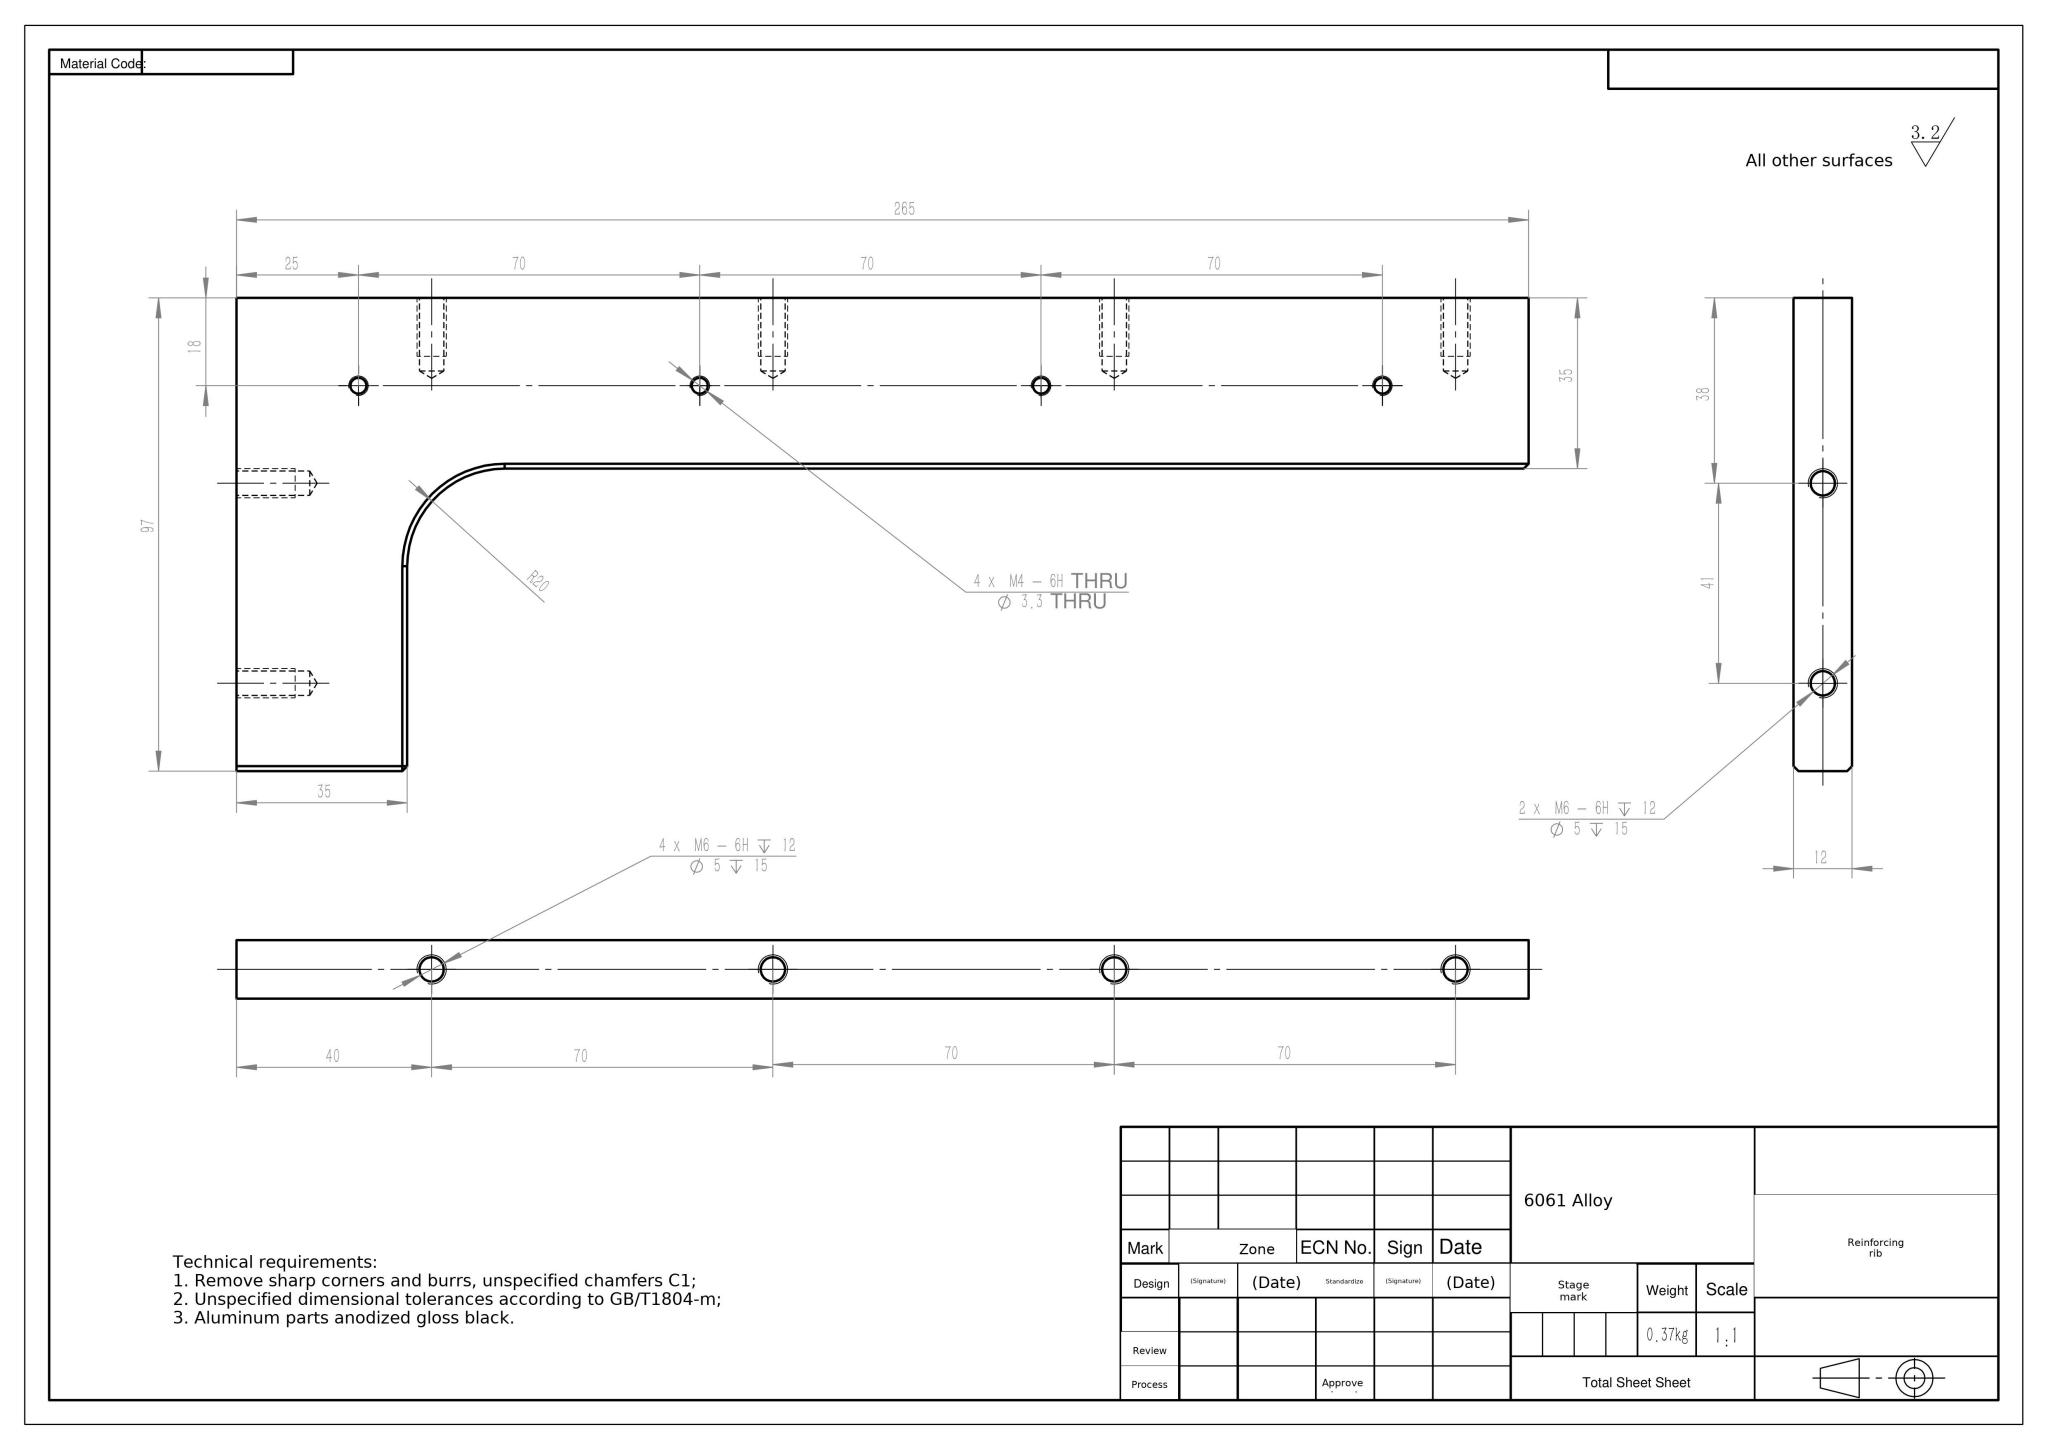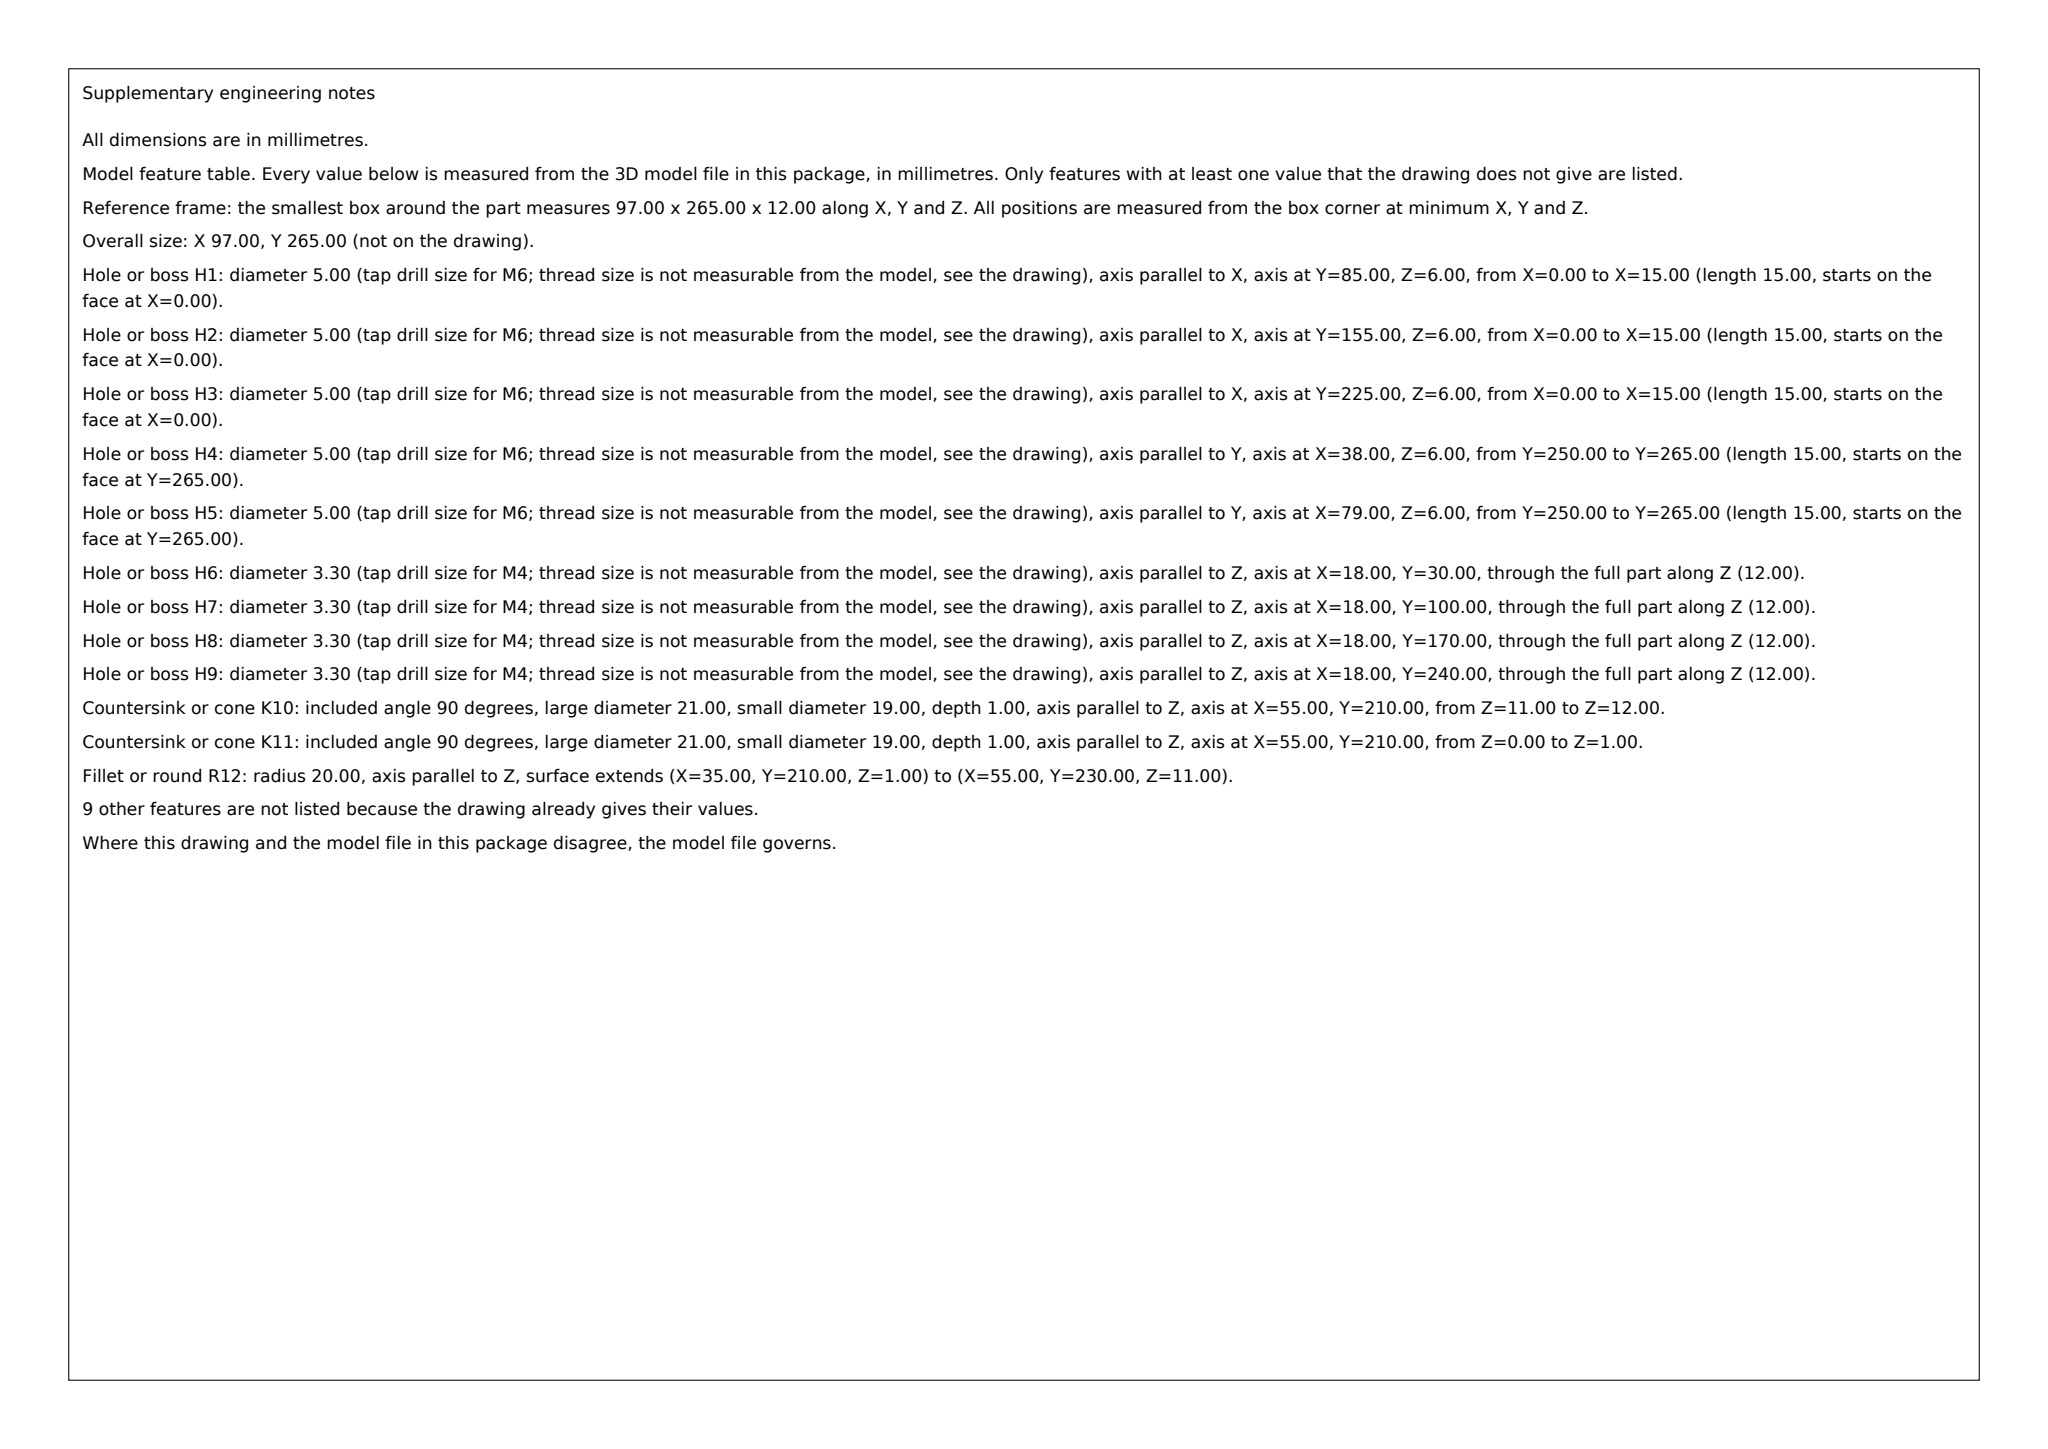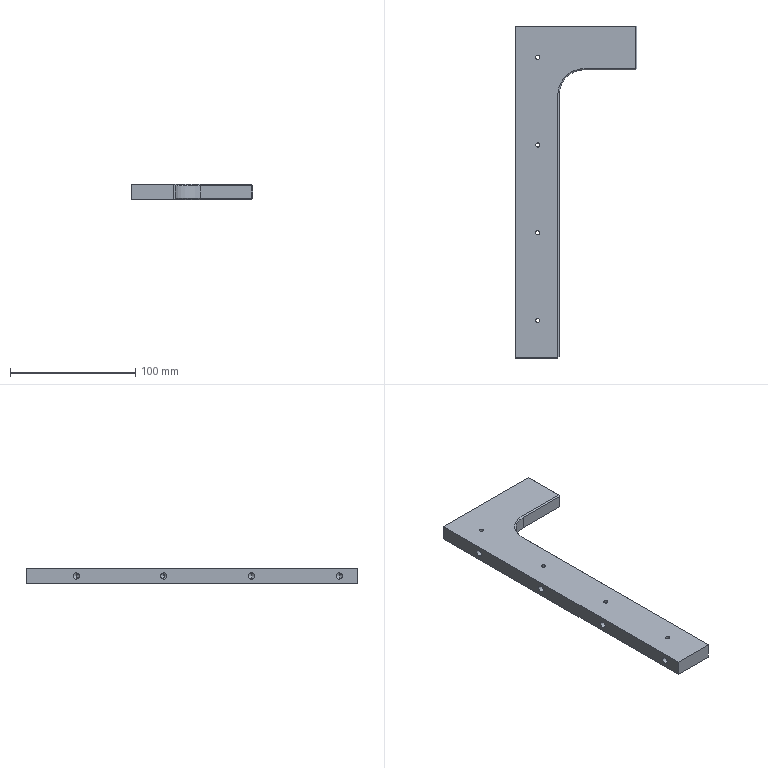Part | SolidWorks | mm | material 6061 Alloy | 1 solid | 53 faces | box 97 x 265 x 12 mm | volume 135804 mm3 | cylinder 21 | plane 18 | cone 14 | commonest cylinder face diameters 5 x12 3.3 x8 40 x1
build123d program:
from build123d import *

# Parameters (mm, degrees)
BOSS_EXTRUDE1_DEPTH   = 12
M6_TAPPED_HOLE1_D     = 5
M6_TAPPED_HOLE1_DEPTH = 15
M6_TAPPED_HOLE1_TIP   = 1.502
M6_TAPPED_HOLE2_D     = 5
M6_TAPPED_HOLE2_DEPTH = 15
M6_TAPPED_HOLE2_TIP   = 1.502
M4_TAPPED_HOLE1_D     = 3.3
FILLET1_R             = 20
CHAMFER1_SIZE         = 1


with BuildPart() as part:
    # Sketch1 → Boss-Extrude1 (new body)
    with BuildSketch(Plane.XY):
        Polygon((97, 230), (35, 230), (35, 0), (0, 0), (0, 265), (97, 265), align=None)
    extrude(amount=BOSS_EXTRUDE1_DEPTH)

    # M6 Tapped Hole1
    with Locations(Plane(origin=(0, 265, 0), x_dir=(1, 0, 0), z_dir=(0, 1, 0))):
        with Locations((38, -6), (79, -6)):
            Hole(M6_TAPPED_HOLE1_D / 2, depth=M6_TAPPED_HOLE1_DEPTH)
            with Locations((0, 0, -(M6_TAPPED_HOLE1_DEPTH + M6_TAPPED_HOLE1_TIP / 2))):  # 118° drill point
                Cone(0, M6_TAPPED_HOLE1_D / 2, M6_TAPPED_HOLE1_TIP, mode=Mode.SUBTRACT)

    # M6 Tapped Hole2
    with Locations(Plane.ZY):
        with Locations((6, 225), (6, 155), (6, 85), (6, 15)):
            Hole(M6_TAPPED_HOLE2_D / 2, depth=M6_TAPPED_HOLE2_DEPTH)
            with Locations((0, 0, -(M6_TAPPED_HOLE2_DEPTH + M6_TAPPED_HOLE2_TIP / 2))):  # 118° drill point
                Cone(0, M6_TAPPED_HOLE2_D / 2, M6_TAPPED_HOLE2_TIP, mode=Mode.SUBTRACT)

    # M4 Tapped Hole1 (through all)
    with Locations(Plane.XY.offset(12)):
        with Locations((18, 240), (18, 170), (18, 100), (18, 30)):
            Hole(M4_TAPPED_HOLE1_D / 2)

    # Fillet1
    fillet1_edges = [part.edges().sort_by_distance(p)[0] for p in [
        (35, 230, 6),
    ]]
    fillet(fillet1_edges, radius=FILLET1_R)

    # Chamfer1
    chamfer1_edges = [part.edges().sort_by_distance(p)[0] for p in [
        (97, 230, 6),
        (35, 0, 6),
        (35, 105, 12),
        (97, 247.5, 12),
        (76, 230, 0),
        (76, 230, 12),
        (40.858, 224.142, 0),
        (40.858, 224.142, 12),
        (97, 247.5, 0),
        (35, 105, 0),
    ]]
    chamfer(chamfer1_edges, length=CHAMFER1_SIZE)


solid = part.part